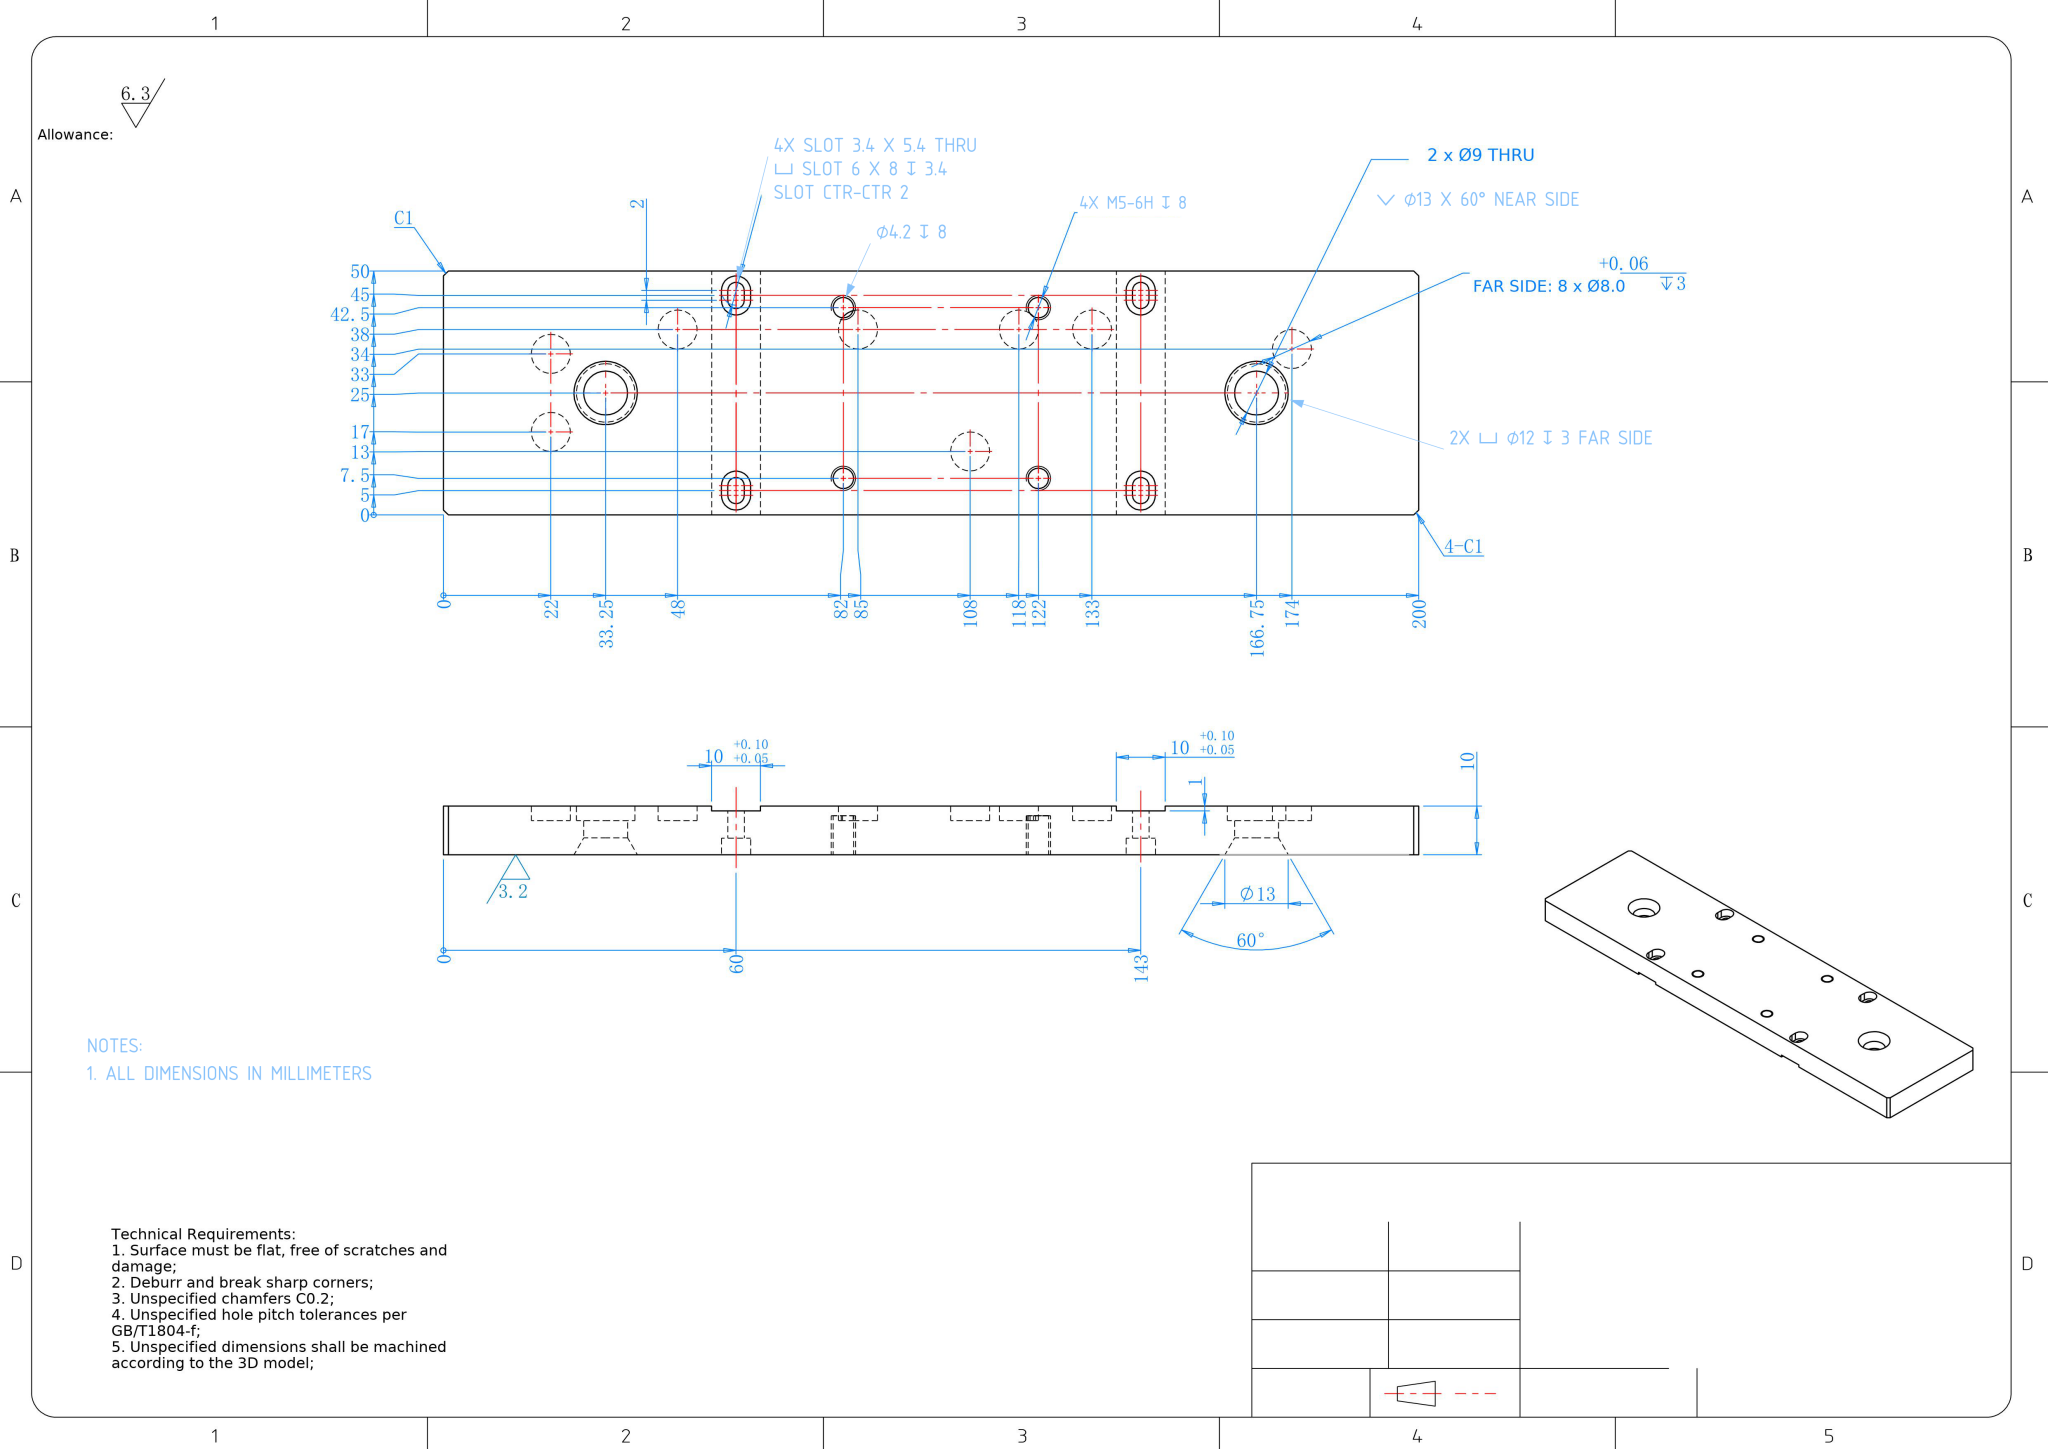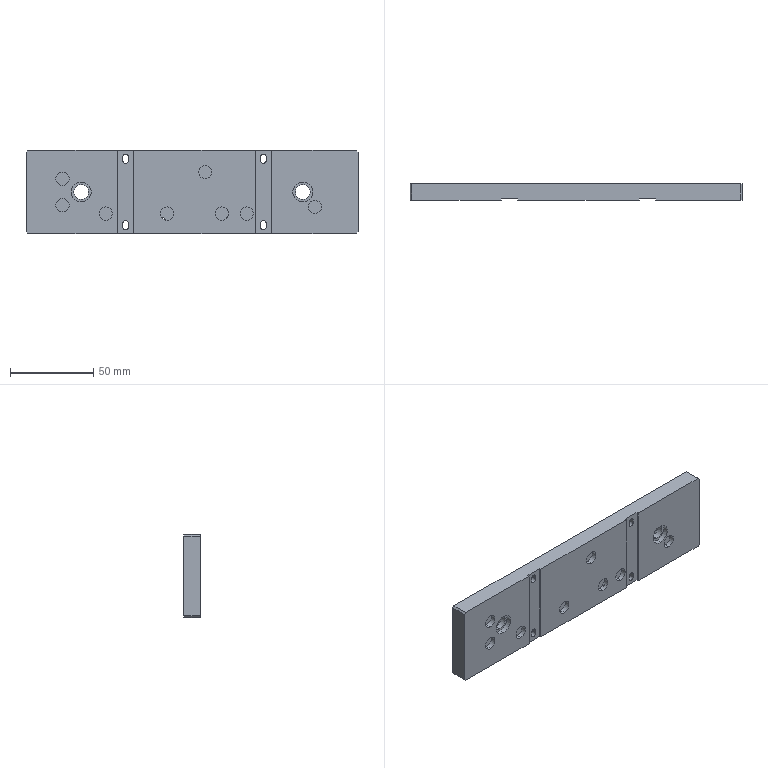Part | NX | mm | 1 solid | 112 faces | box 200 x 10 x 50 mm | volume 94634 mm3 | cylinder 56 | plane 52 | cone 4 | commonest cylinder face diameters 8 x16 6 x12 3.4 x12 4.2 x8 12 x4 9 x4